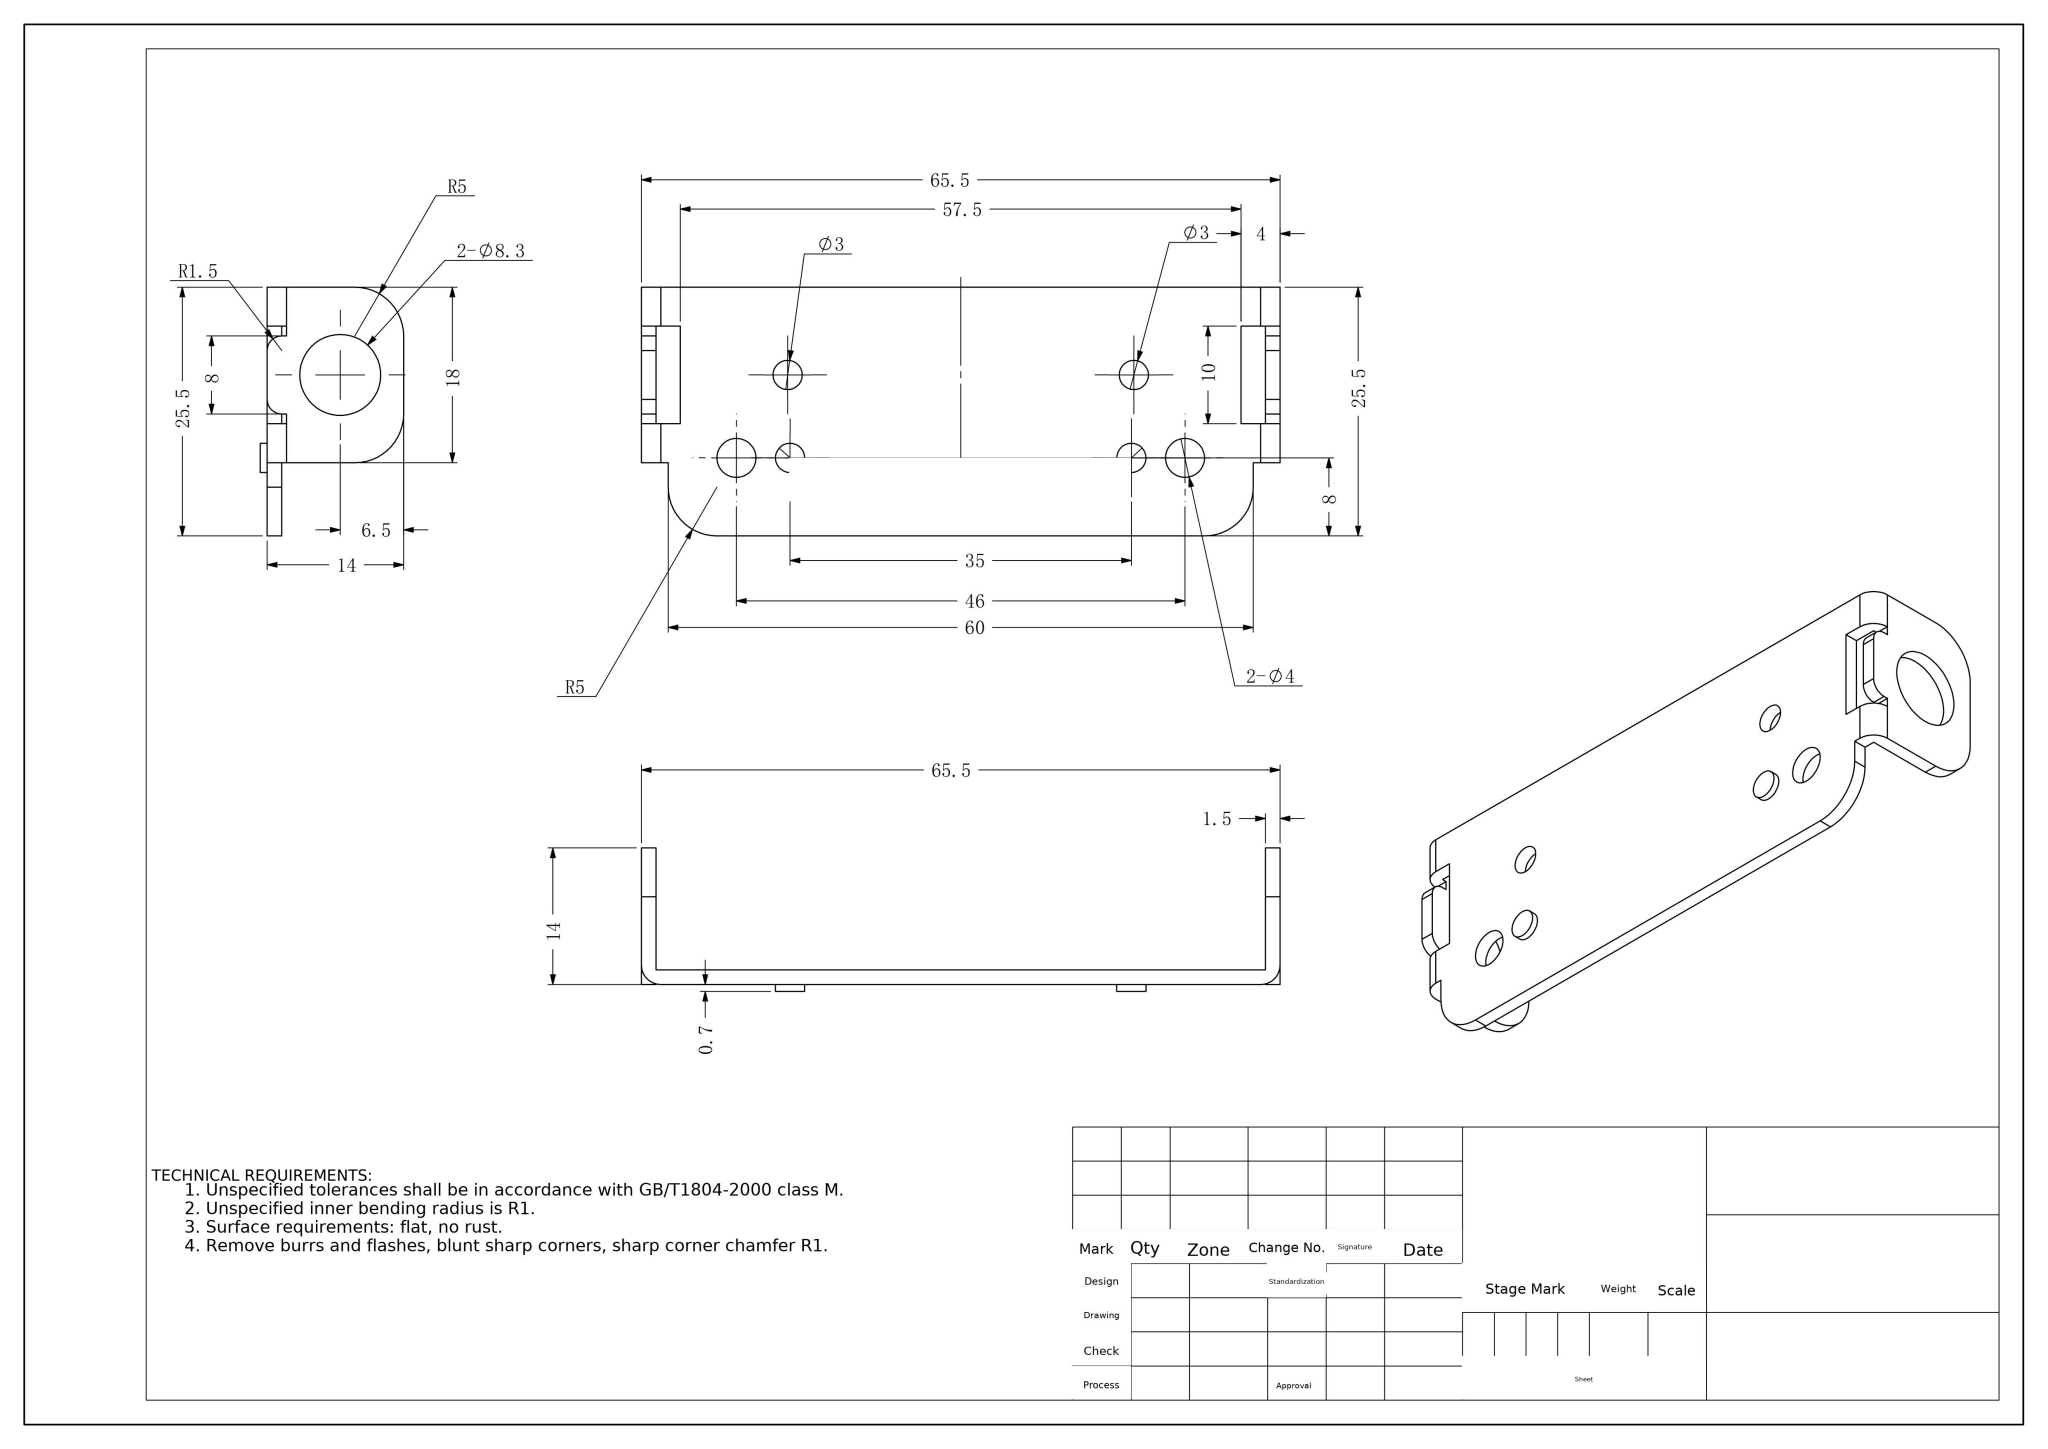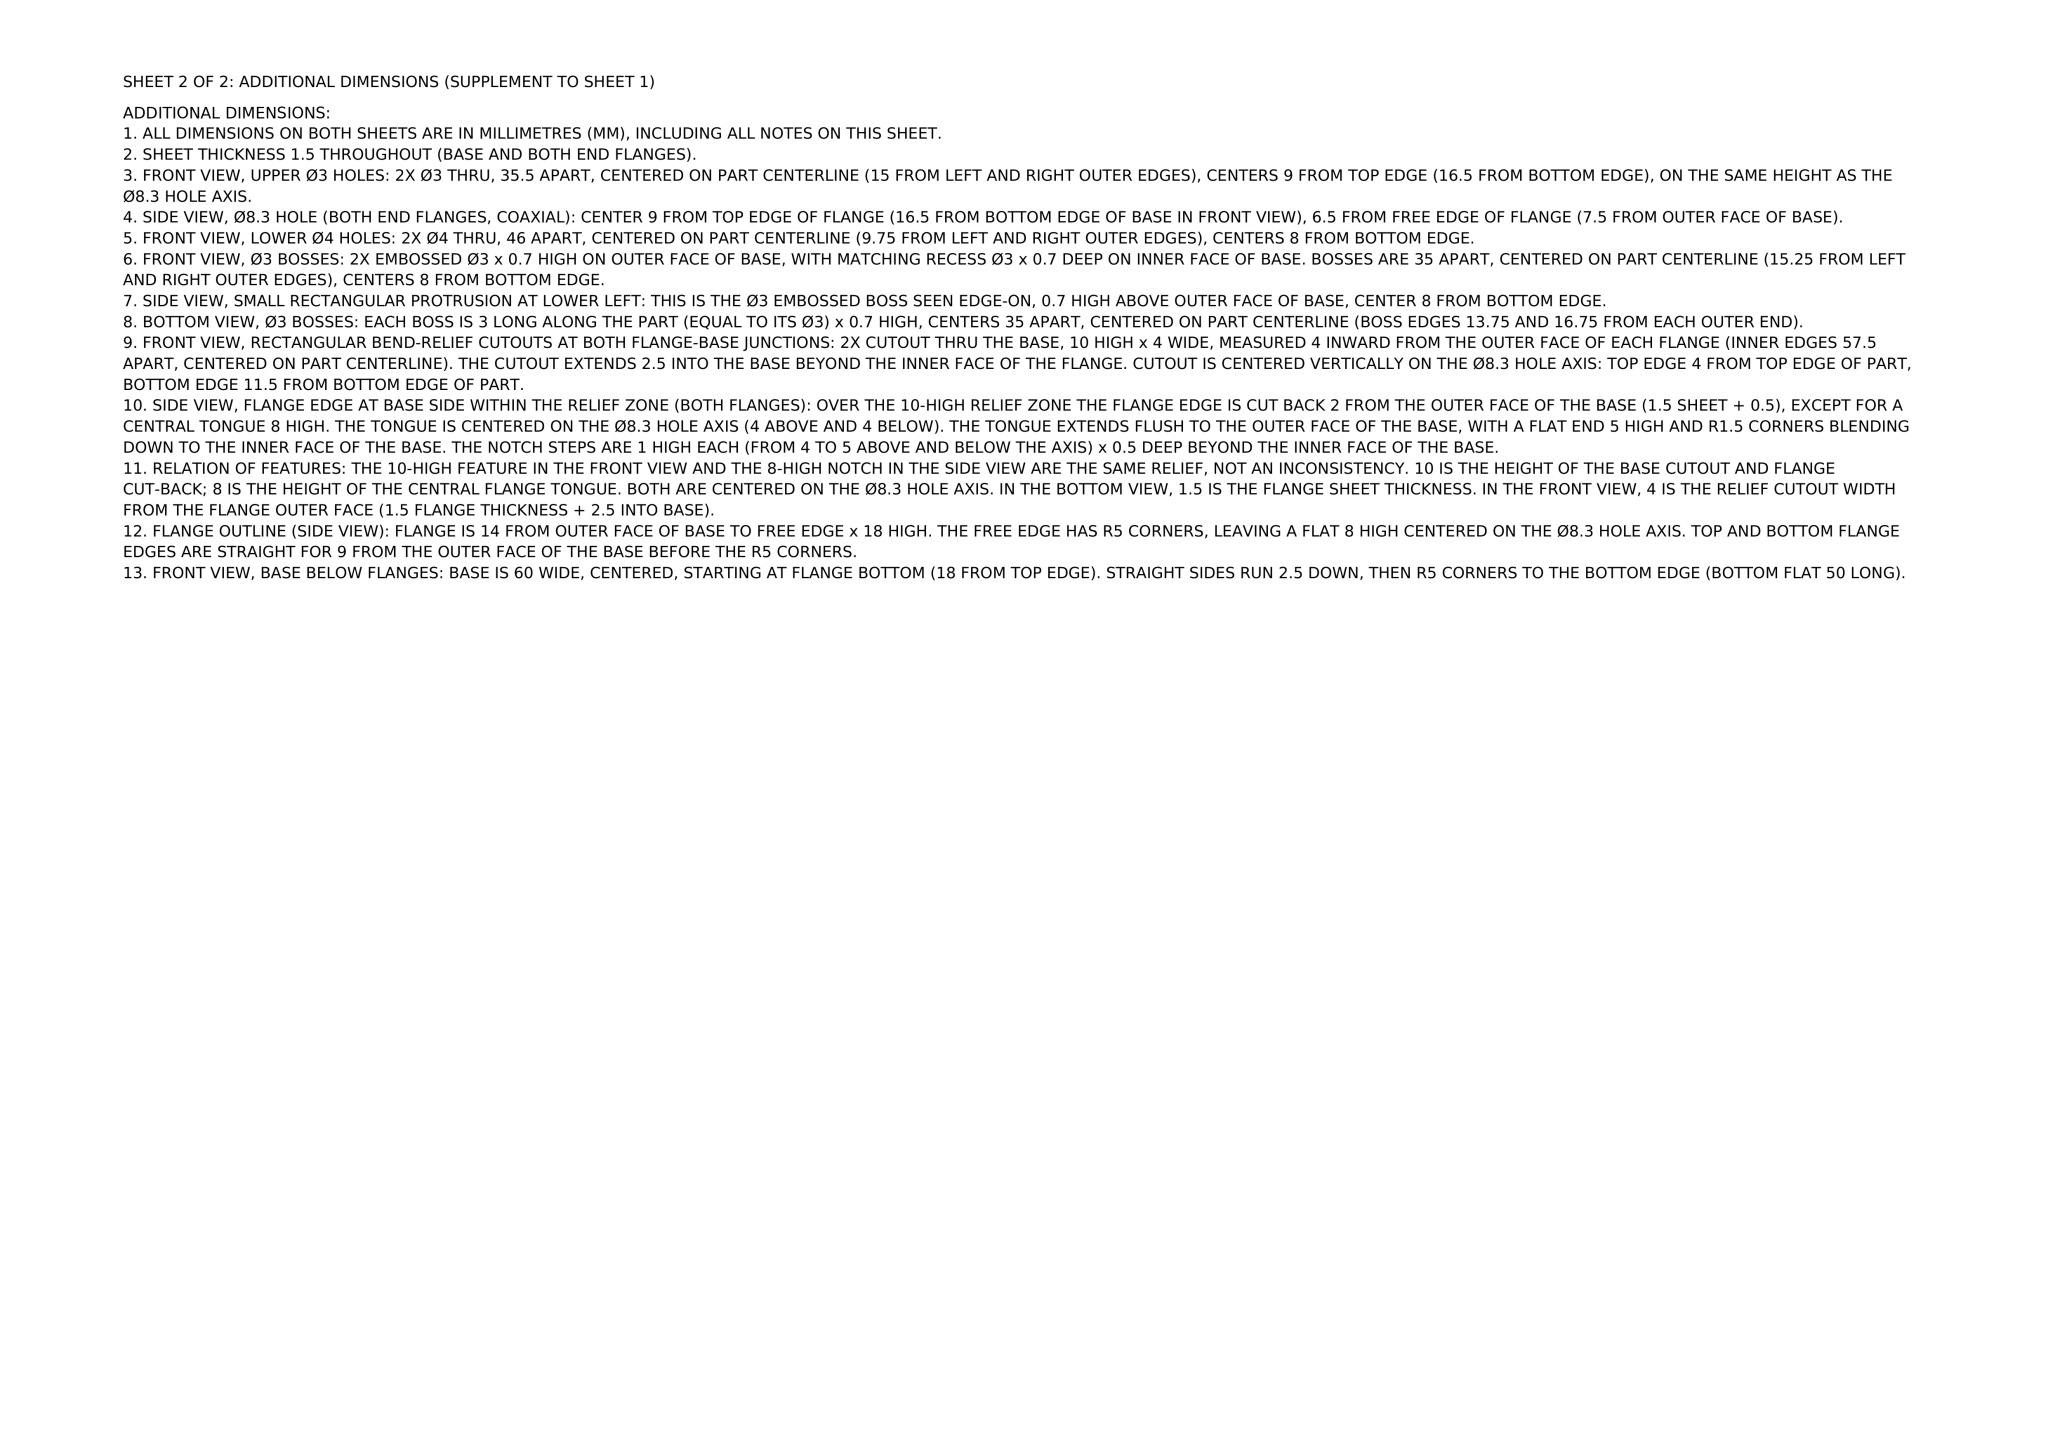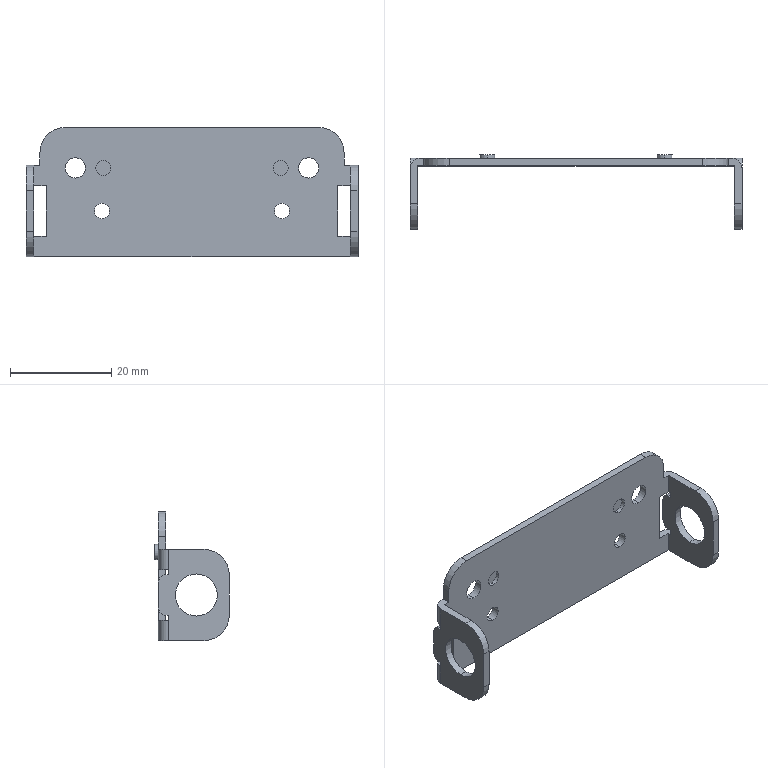Part | NX | mm | 1 solid | 68 faces | box 65.5 x 14.7 x 25.5 mm | volume 2745 mm3 | cylinder 34 | plane 34 | commonest cylinder face diameters 3 x16 10 x6 4 x4 8.3 x4 4.004 x4